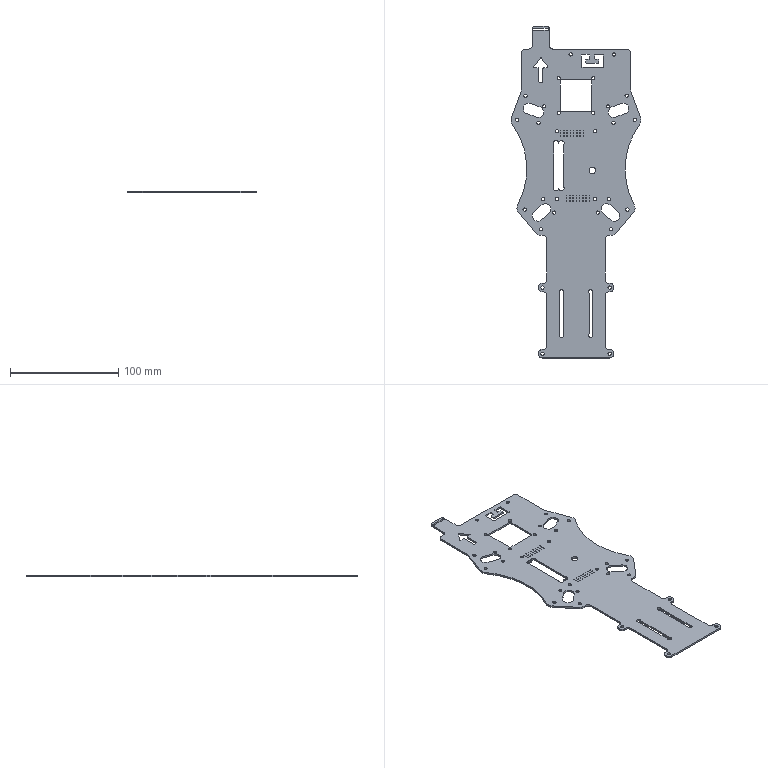Component | SolidWorks | UpperPlate-3 | 1 solid | 403 faces | volume 33833 mm3 | plane 251 | cylinder 152 | commonest cylinder face diameters 3 x52 1 x20 6 x14 4 x12 10 x12 8 x8 13 x8 2 x7